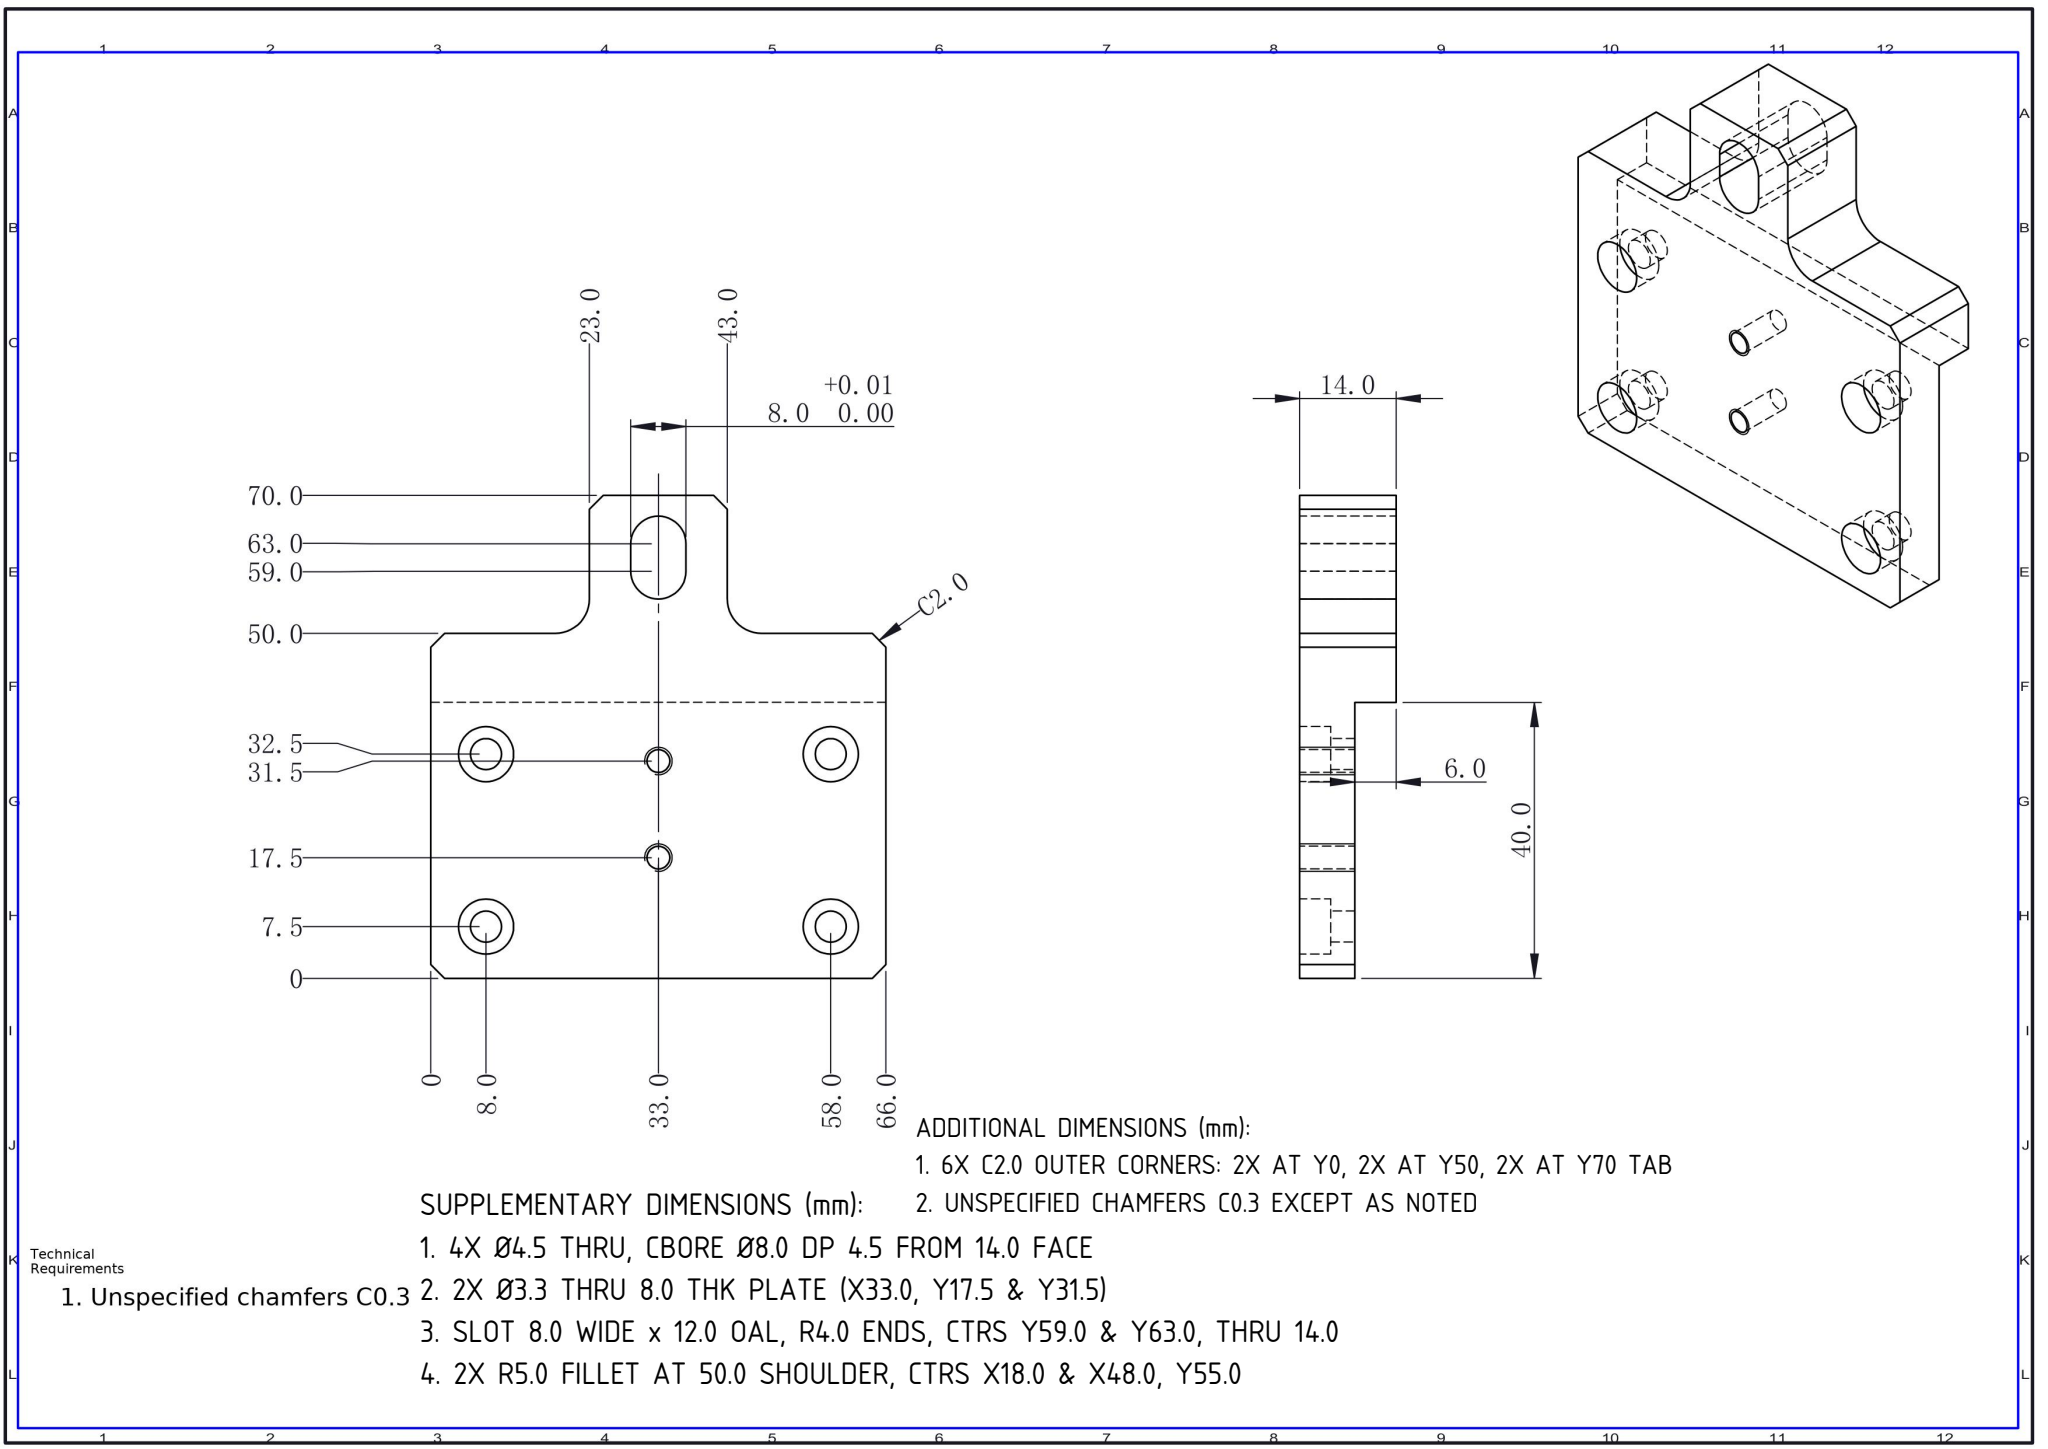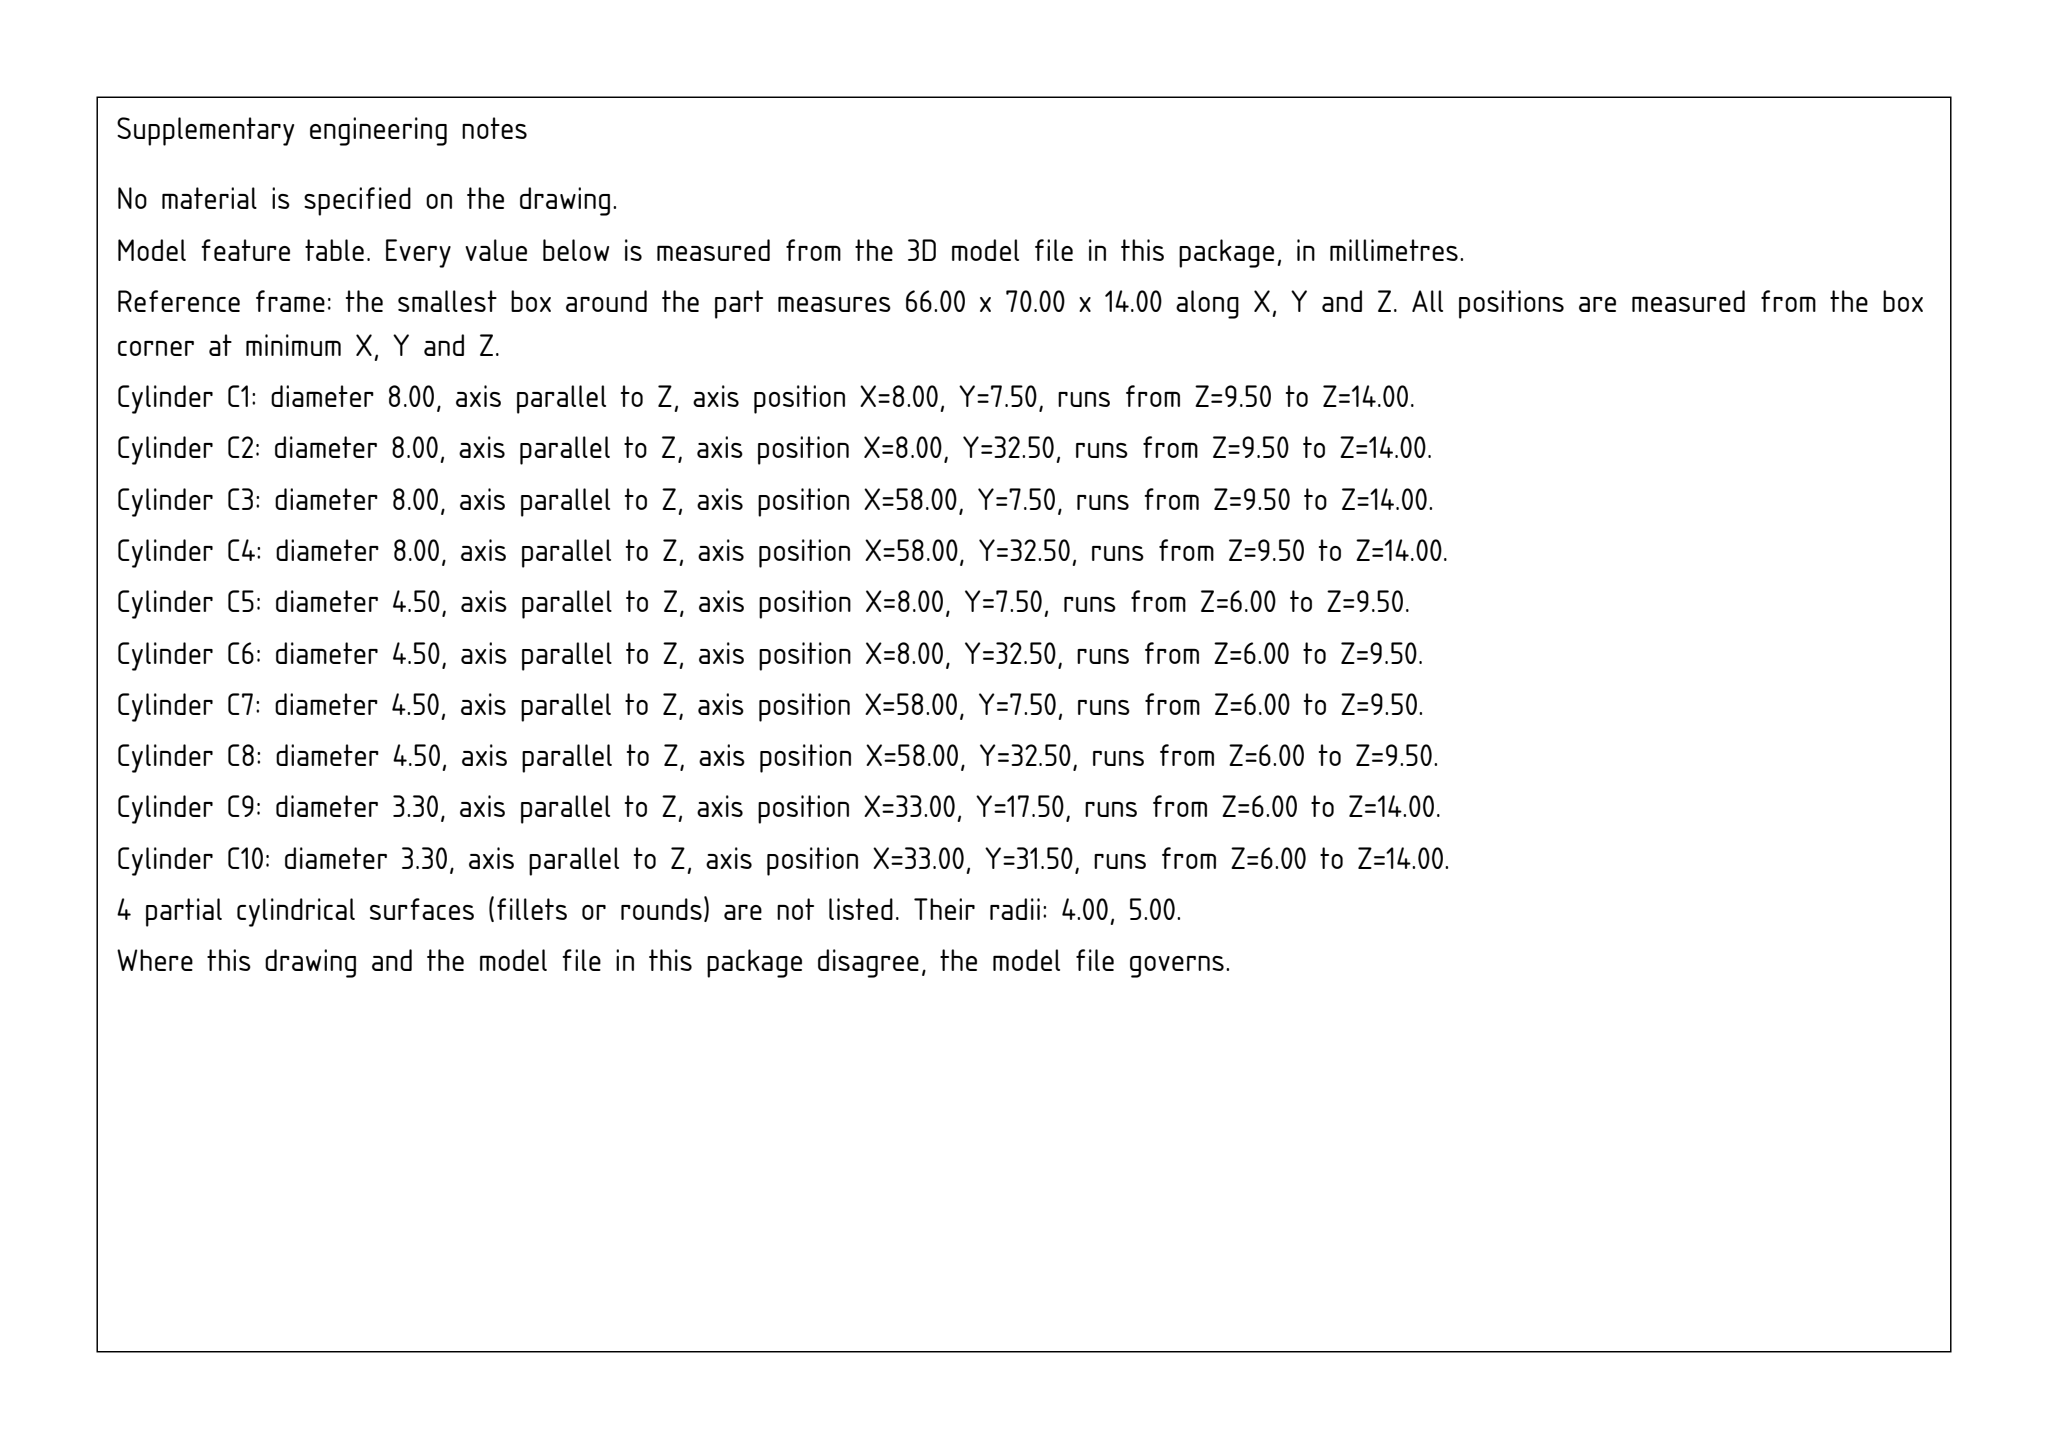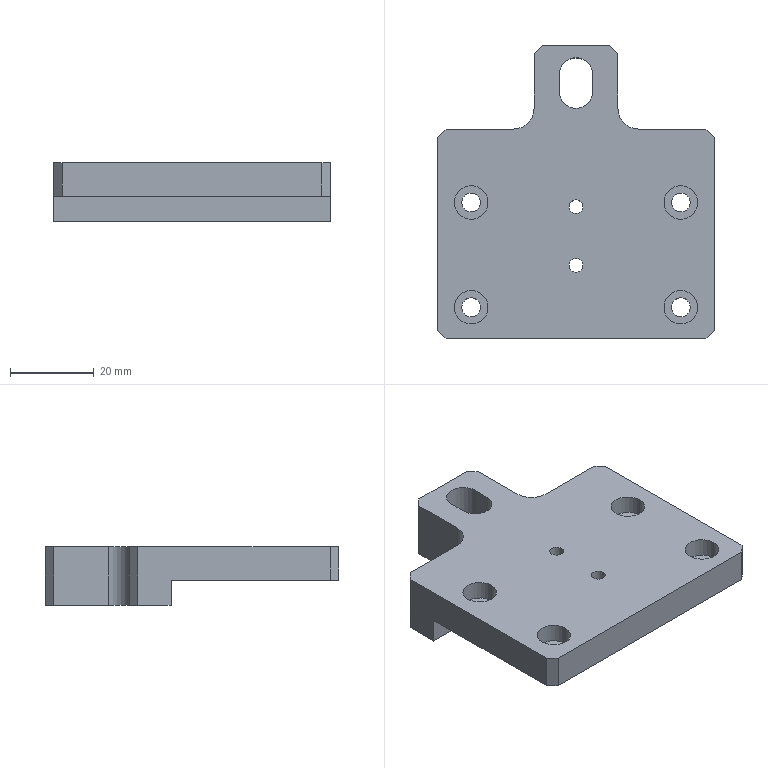Part | SolidWorks | mm | 1 solid | 48 faces | box 66 x 70 x 14 mm | volume 33550 mm3 | cylinder 24 | plane 24 | commonest cylinder face diameters 8 x10 4.5 x8 3.3 x4 10 x2